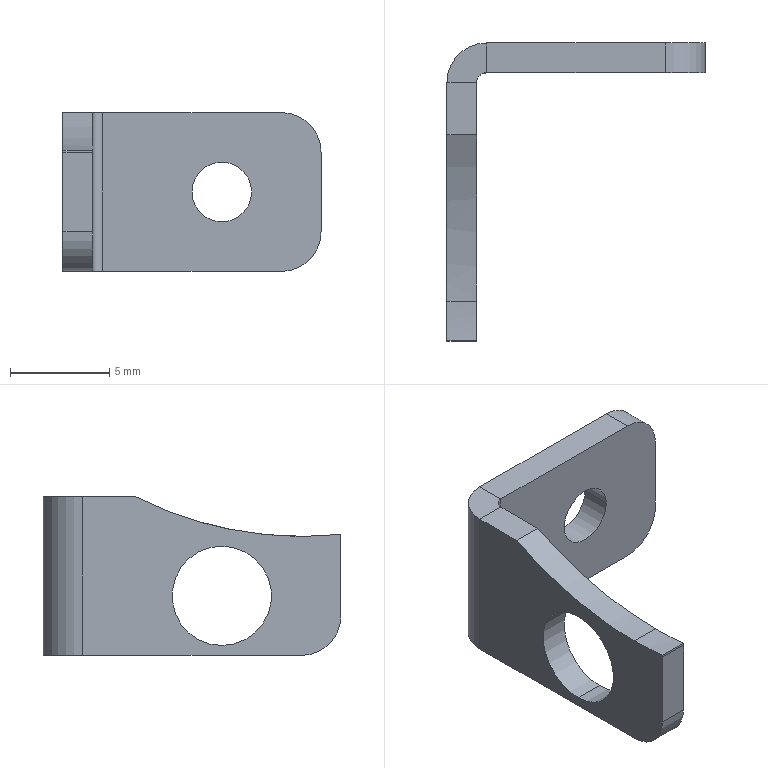Component | SolidWorks | ZHDJ-A0017-1 | 1 solid | 24 faces | box 13 x 15 x 8 mm | volume 245 mm3 | cylinder 12 | plane 12 | commonest cylinder face diameters 4 x5 37 x2 5 x2 3 x2 1 x1
STEP:
#1=COLOUR_RGB('',0.7922,0.8196,0.9333);
#2=FILL_AREA_STYLE_COLOUR('',#1);
#3=FILL_AREA_STYLE('',(#2));
#4=SURFACE_STYLE_FILL_AREA(#3);
#5=SURFACE_SIDE_STYLE('',(#4));
#6=SURFACE_STYLE_USAGE(.BOTH.,#5);
#7=PRESENTATION_STYLE_ASSIGNMENT((#6));
#8=CARTESIAN_POINT('',(0.2559,-0.07863,6.874));
#9=VERTEX_POINT('',#8);
#10=CARTESIAN_POINT('',(0.2559,0.,6.87));
#11=VERTEX_POINT('',#10);
#12=CARTESIAN_POINT('',(0.2559,0.,7.598));
#13=DIRECTION('',(1.,0.,-0.));
#14=DIRECTION('',(0.,-0.,1.));
#15=AXIS2_PLACEMENT_3D('',#12,#13,#14);
#16=CIRCLE('',#15,0.7283);
#17=EDGE_CURVE('',#9,#11,#16,.T.);
#18=ORIENTED_EDGE('',*,*,#17,.T.);
#19=CARTESIAN_POINT('',(0.1969,0.,6.87));
#20=VERTEX_POINT('',#19);
#21=CARTESIAN_POINT('',(0.7087,0.,6.87));
#22=DIRECTION('',(-1.,-0.,0.));
#23=VECTOR('',#22,39.37);
#24=LINE('',#21,#23);
#25=EDGE_CURVE('',#11,#20,#24,.T.);
#26=ORIENTED_EDGE('',*,*,#25,.T.);
#27=CARTESIAN_POINT('',(0.1969,-0.07862,6.874));
#28=VERTEX_POINT('',#27);
#29=CARTESIAN_POINT('',(0.1969,0.,6.87));
#30=CARTESIAN_POINT('',(0.1968,-0.02626,6.87));
#31=CARTESIAN_POINT('',(0.1968,-0.05252,6.872));
#32=CARTESIAN_POINT('',(0.1969,-0.07862,6.874));
#33=B_SPLINE_CURVE_WITH_KNOTS('',3,(#29,#30,#31,#32),.UNSPECIFIED.,.F.,.F.,(4,4),(0.8127,1.),.UNSPECIFIED.);
#34=EDGE_CURVE('',#20,#28,#33,.T.);
#35=ORIENTED_EDGE('',*,*,#34,.T.);
#36=CARTESIAN_POINT('',(0.4528,-0.07863,6.874));
#37=DIRECTION('',(1.,0.,-0.));
#38=VECTOR('',#37,39.37);
#39=LINE('',#36,#38);
#40=EDGE_CURVE('',#28,#9,#39,.T.);
#41=ORIENTED_EDGE('',*,*,#40,.T.);
#42=EDGE_LOOP('',(#18,#26,#35,#41));
#43=FACE_OUTER_BOUND('',#42,.T.);
#44=CARTESIAN_POINT('',(0.7087,0.,7.598));
#45=DIRECTION('',(-1.,-0.,0.));
#46=DIRECTION('',(0.,0.,-1.));
#47=AXIS2_PLACEMENT_3D('',#44,#45,#46);
#48=CYLINDRICAL_SURFACE('',#47,0.7283);
#49=ADVANCED_FACE('',(#43),#48,.F.);
#50=CARTESIAN_POINT('',(0.2559,0.1575,6.654));
#51=VERTEX_POINT('',#50);
#52=CARTESIAN_POINT('',(0.2559,0.1575,6.85));
#53=VERTEX_POINT('',#52);
#54=CARTESIAN_POINT('',(0.2559,0.1575,6.752));
#55=DIRECTION('',(1.,0.,-0.));
#56=DIRECTION('',(0.,0.,1.));
#57=AXIS2_PLACEMENT_3D('',#54,#55,#56);
#58=CIRCLE('',#57,0.09843);
#59=EDGE_CURVE('',#51,#53,#58,.T.);
#60=ORIENTED_EDGE('',*,*,#59,.T.);
#61=CARTESIAN_POINT('',(0.1969,0.1575,6.85));
#62=VERTEX_POINT('',#61);
#63=CARTESIAN_POINT('',(0.5906,0.1575,6.85));
#64=DIRECTION('',(-1.,-0.,0.));
#65=VECTOR('',#64,39.37);
#66=LINE('',#63,#65);
#67=EDGE_CURVE('',#53,#62,#66,.T.);
#68=ORIENTED_EDGE('',*,*,#67,.T.);
#69=CARTESIAN_POINT('',(0.1969,0.1575,6.654));
#70=VERTEX_POINT('',#69);
#71=CARTESIAN_POINT('',(0.1969,0.1575,6.752));
#72=DIRECTION('',(-1.,-0.,0.));
#73=DIRECTION('',(0.,0.,-1.));
#74=AXIS2_PLACEMENT_3D('',#71,#72,#73);
#75=CIRCLE('',#74,0.09843);
#76=EDGE_CURVE('',#62,#70,#75,.T.);
#77=ORIENTED_EDGE('',*,*,#76,.T.);
#78=CARTESIAN_POINT('',(0.5906,0.1575,6.654));
#79=DIRECTION('',(-1.,-0.,0.));
#80=VECTOR('',#79,39.37);
#81=LINE('',#78,#80);
#82=EDGE_CURVE('',#51,#70,#81,.T.);
#83=ORIENTED_EDGE('',*,*,#82,.F.);
#84=EDGE_LOOP('',(#60,#68,#77,#83));
#85=FACE_OUTER_BOUND('',#84,.T.);
#86=CARTESIAN_POINT('',(0.5906,0.1575,6.752));
#87=DIRECTION('',(-1.,-0.,0.));
#88=DIRECTION('',(0.,0.,-1.));
#89=AXIS2_PLACEMENT_3D('',#86,#87,#88);
#90=CYLINDRICAL_SURFACE('',#89,0.09843);
#91=ADVANCED_FACE('',(#85),#90,.F.);
#92=CARTESIAN_POINT('',(0.5709,0.5118,6.791));
#93=VERTEX_POINT('',#92);
#94=CARTESIAN_POINT('',(0.4528,0.5118,6.791));
#95=VERTEX_POINT('',#94);
#96=CARTESIAN_POINT('',(0.5118,0.5118,6.791));
#97=DIRECTION('',(0.,-1.,0.));
#98=DIRECTION('',(-1.,0.,0.));
#99=AXIS2_PLACEMENT_3D('',#96,#97,#98);
#100=CIRCLE('',#99,0.05906);
#101=EDGE_CURVE('',#93,#95,#100,.T.);
#102=ORIENTED_EDGE('',*,*,#101,.F.);
#103=CARTESIAN_POINT('',(0.5709,0.4528,6.791));
#104=VERTEX_POINT('',#103);
#105=CARTESIAN_POINT('',(0.5709,0.8465,6.791));
#106=DIRECTION('',(0.,-1.,0.));
#107=VECTOR('',#106,39.37);
#108=LINE('',#105,#107);
#109=EDGE_CURVE('',#93,#104,#108,.T.);
#110=ORIENTED_EDGE('',*,*,#109,.T.);
#111=CARTESIAN_POINT('',(0.4528,0.4528,6.791));
#112=VERTEX_POINT('',#111);
#113=CARTESIAN_POINT('',(0.5118,0.4528,6.791));
#114=DIRECTION('',(0.,-1.,0.));
#115=DIRECTION('',(-1.,0.,0.));
#116=AXIS2_PLACEMENT_3D('',#113,#114,#115);
#117=CIRCLE('',#116,0.05906);
#118=EDGE_CURVE('',#104,#112,#117,.T.);
#119=ORIENTED_EDGE('',*,*,#118,.T.);
#120=CARTESIAN_POINT('',(0.4528,0.8465,6.791));
#121=DIRECTION('',(0.,-1.,0.));
#122=VECTOR('',#121,39.37);
#123=LINE('',#120,#122);
#124=EDGE_CURVE('',#95,#112,#123,.T.);
#125=ORIENTED_EDGE('',*,*,#124,.F.);
#126=EDGE_LOOP('',(#102,#110,#119,#125));
#127=FACE_OUTER_BOUND('',#126,.T.);
#128=CARTESIAN_POINT('',(0.5118,0.8465,6.791));
#129=DIRECTION('',(0.,-1.,0.));
#130=DIRECTION('',(-1.,0.,0.));
#131=AXIS2_PLACEMENT_3D('',#128,#129,#130);
#132=CYLINDRICAL_SURFACE('',#131,0.05906);
#133=ADVANCED_FACE('',(#127),#132,.F.);
#134=CARTESIAN_POINT('',(0.1969,0.1575,6.752));
#135=DIRECTION('',(-1.,-0.,0.));
#136=DIRECTION('',(0.,0.,-1.));
#137=AXIS2_PLACEMENT_3D('',#134,#135,#136);
#138=CIRCLE('',#137,0.09843);
#139=EDGE_CURVE('',#70,#62,#138,.T.);
#140=ORIENTED_EDGE('',*,*,#139,.F.);
#141=ORIENTED_EDGE('',*,*,#76,.F.);
#142=EDGE_LOOP('',(#140,#141));
#143=FACE_BOUND('',#142,.T.);
#144=CARTESIAN_POINT('',(0.1969,0.3295,6.949));
#145=VERTEX_POINT('',#144);
#146=CARTESIAN_POINT('',(0.1969,0.3295,6.949));
#147=CARTESIAN_POINT('',(0.1968,0.2786,6.923));
#148=CARTESIAN_POINT('',(0.1968,0.2248,6.903));
#149=CARTESIAN_POINT('',(0.1968,0.1139,6.877));
#150=CARTESIAN_POINT('',(0.1968,0.05698,6.87));
#151=CARTESIAN_POINT('',(0.1969,0.,6.87));
#152=B_SPLINE_CURVE_WITH_KNOTS('',3,(#146,#147,#148,#149,#150,#151),.UNSPECIFIED.,.F.,.F.,(4,2,4),(0.,0.4064,0.8127),.UNSPECIFIED.);
#153=EDGE_CURVE('',#145,#20,#152,.T.);
#154=ORIENTED_EDGE('',*,*,#153,.F.);
#155=CARTESIAN_POINT('',(0.1969,0.4331,6.949));
#156=VERTEX_POINT('',#155);
#157=CARTESIAN_POINT('',(0.1969,0.4528,6.949));
#158=DIRECTION('',(-0.,1.,0.));
#159=VECTOR('',#158,39.37);
#160=LINE('',#157,#159);
#161=EDGE_CURVE('',#145,#156,#160,.T.);
#162=ORIENTED_EDGE('',*,*,#161,.T.);
#163=CARTESIAN_POINT('',(0.1969,0.4331,6.634));
#164=VERTEX_POINT('',#163);
#165=CARTESIAN_POINT('',(0.1969,0.4331,6.949));
#166=DIRECTION('',(0.,-0.,1.));
#167=VECTOR('',#166,39.37);
#168=LINE('',#165,#167);
#169=EDGE_CURVE('',#164,#156,#168,.T.);
#170=ORIENTED_EDGE('',*,*,#169,.F.);
#171=CARTESIAN_POINT('',(0.1969,0.,6.634));
#172=VERTEX_POINT('',#171);
#173=CARTESIAN_POINT('',(0.1969,0.4528,6.634));
#174=DIRECTION('',(0.,-1.,0.));
#175=VECTOR('',#174,39.37);
#176=LINE('',#173,#175);
#177=EDGE_CURVE('',#164,#172,#176,.T.);
#178=ORIENTED_EDGE('',*,*,#177,.T.);
#179=CARTESIAN_POINT('',(0.1969,-0.07874,6.713));
#180=VERTEX_POINT('',#179);
#181=CARTESIAN_POINT('',(0.1969,0.,6.713));
#182=DIRECTION('',(-1.,-0.,0.));
#183=DIRECTION('',(0.,-0.,1.));
#184=AXIS2_PLACEMENT_3D('',#181,#182,#183);
#185=CIRCLE('',#184,0.07874);
#186=EDGE_CURVE('',#172,#180,#185,.T.);
#187=ORIENTED_EDGE('',*,*,#186,.T.);
#188=CARTESIAN_POINT('',(0.1969,-0.07874,6.87));
#189=VERTEX_POINT('',#188);
#190=CARTESIAN_POINT('',(0.1969,-0.07874,6.791));
#191=DIRECTION('',(0.,-0.,1.));
#192=VECTOR('',#191,39.37);
#193=LINE('',#190,#192);
#194=EDGE_CURVE('',#180,#189,#193,.T.);
#195=ORIENTED_EDGE('',*,*,#194,.T.);
#196=CARTESIAN_POINT('',(0.1969,0.,6.87));
#197=DIRECTION('',(-1.,-0.,0.));
#198=DIRECTION('',(0.,0.,1.));
#199=AXIS2_PLACEMENT_3D('',#196,#197,#198);
#200=CIRCLE('',#199,0.07874);
#201=EDGE_CURVE('',#189,#28,#200,.T.);
#202=ORIENTED_EDGE('',*,*,#201,.T.);
#203=ORIENTED_EDGE('',*,*,#34,.F.);
#204=EDGE_LOOP('',(#154,#162,#170,#178,#187,#195,#202,#203));
#205=FACE_OUTER_BOUND('',#204,.T.);
#206=CARTESIAN_POINT('',(0.1969,0.4528,6.791));
#207=DIRECTION('',(1.,0.,-0.));
#208=DIRECTION('',(0.,-0.,1.));
#209=AXIS2_PLACEMENT_3D('',#206,#207,#208);
#210=PLANE('',#209);
#211=ADVANCED_FACE('',(#143,#205),#210,.F.);
#212=CARTESIAN_POINT('',(0.5118,0.5118,6.791));
#213=DIRECTION('',(0.,-1.,0.));
#214=DIRECTION('',(-1.,0.,0.));
#215=AXIS2_PLACEMENT_3D('',#212,#213,#214);
#216=CIRCLE('',#215,0.05906);
#217=EDGE_CURVE('',#95,#93,#216,.T.);
#218=ORIENTED_EDGE('',*,*,#217,.T.);
#219=ORIENTED_EDGE('',*,*,#101,.T.);
#220=EDGE_LOOP('',(#218,#219));
#221=FACE_BOUND('',#220,.T.);
#222=CARTESIAN_POINT('',(0.7087,0.5118,6.713));
#223=VERTEX_POINT('',#222);
#224=CARTESIAN_POINT('',(0.7087,0.5118,6.87));
#225=VERTEX_POINT('',#224);
#226=CARTESIAN_POINT('',(0.7087,0.5118,6.634));
#227=DIRECTION('',(0.,-0.,1.));
#228=VECTOR('',#227,39.37);
#229=LINE('',#226,#228);
#230=EDGE_CURVE('',#223,#225,#229,.T.);
#231=ORIENTED_EDGE('',*,*,#230,.F.);
#232=CARTESIAN_POINT('',(0.6299,0.5118,6.634));
#233=VERTEX_POINT('',#232);
#234=CARTESIAN_POINT('',(0.6299,0.5118,6.713));
#235=DIRECTION('',(-0.,1.,0.));
#236=DIRECTION('',(-1.,0.,0.));
#237=AXIS2_PLACEMENT_3D('',#234,#235,#236);
#238=CIRCLE('',#237,0.07874);
#239=EDGE_CURVE('',#223,#233,#238,.T.);
#240=ORIENTED_EDGE('',*,*,#239,.T.);
#241=CARTESIAN_POINT('',(0.2756,0.5118,6.634));
#242=VERTEX_POINT('',#241);
#243=CARTESIAN_POINT('',(0.1969,0.5118,6.634));
#244=DIRECTION('',(1.,0.,-0.));
#245=VECTOR('',#244,39.37);
#246=LINE('',#243,#245);
#247=EDGE_CURVE('',#242,#233,#246,.T.);
#248=ORIENTED_EDGE('',*,*,#247,.F.);
#249=CARTESIAN_POINT('',(0.2756,0.5118,6.949));
#250=VERTEX_POINT('',#249);
#251=CARTESIAN_POINT('',(0.2756,0.5118,6.634));
#252=DIRECTION('',(0.,-0.,1.));
#253=VECTOR('',#252,39.37);
#254=LINE('',#251,#253);
#255=EDGE_CURVE('',#242,#250,#254,.T.);
#256=ORIENTED_EDGE('',*,*,#255,.T.);
#257=CARTESIAN_POINT('',(0.6299,0.5118,6.949));
#258=VERTEX_POINT('',#257);
#259=CARTESIAN_POINT('',(0.1969,0.5118,6.949));
#260=DIRECTION('',(1.,0.,-0.));
#261=VECTOR('',#260,39.37);
#262=LINE('',#259,#261);
#263=EDGE_CURVE('',#250,#258,#262,.T.);
#264=ORIENTED_EDGE('',*,*,#263,.T.);
#265=CARTESIAN_POINT('',(0.6299,0.5118,6.87));
#266=DIRECTION('',(-0.,1.,0.));
#267=DIRECTION('',(-1.,0.,0.));
#268=AXIS2_PLACEMENT_3D('',#265,#266,#267);
#269=CIRCLE('',#268,0.07874);
#270=EDGE_CURVE('',#258,#225,#269,.T.);
#271=ORIENTED_EDGE('',*,*,#270,.T.);
#272=EDGE_LOOP('',(#231,#240,#248,#256,#264,#271));
#273=FACE_OUTER_BOUND('',#272,.T.);
#274=CARTESIAN_POINT('',(0.1969,0.5118,6.634));
#275=DIRECTION('',(0.,-1.,-0.));
#276=DIRECTION('',(-1.,-0.,0.));
#277=AXIS2_PLACEMENT_3D('',#274,#275,#276);
#278=PLANE('',#277);
#279=ADVANCED_FACE('',(#221,#273),#278,.F.);
#280=CARTESIAN_POINT('',(0.5118,0.4528,6.791));
#281=DIRECTION('',(0.,-1.,0.));
#282=DIRECTION('',(-1.,0.,0.));
#283=AXIS2_PLACEMENT_3D('',#280,#281,#282);
#284=CIRCLE('',#283,0.05906);
#285=EDGE_CURVE('',#112,#104,#284,.T.);
#286=ORIENTED_EDGE('',*,*,#285,.F.);
#287=ORIENTED_EDGE('',*,*,#118,.F.);
#288=EDGE_LOOP('',(#286,#287));
#289=FACE_BOUND('',#288,.T.);
#290=CARTESIAN_POINT('',(0.2756,0.4528,6.634));
#291=VERTEX_POINT('',#290);
#292=CARTESIAN_POINT('',(0.6299,0.4528,6.634));
#293=VERTEX_POINT('',#292);
#294=CARTESIAN_POINT('',(0.1969,0.4528,6.634));
#295=DIRECTION('',(1.,0.,-0.));
#296=VECTOR('',#295,39.37);
#297=LINE('',#294,#296);
#298=EDGE_CURVE('',#291,#293,#297,.T.);
#299=ORIENTED_EDGE('',*,*,#298,.T.);
#300=CARTESIAN_POINT('',(0.7087,0.4528,6.713));
#301=VERTEX_POINT('',#300);
#302=CARTESIAN_POINT('',(0.6299,0.4528,6.713));
#303=DIRECTION('',(0.,-1.,0.));
#304=DIRECTION('',(-1.,0.,0.));
#305=AXIS2_PLACEMENT_3D('',#302,#303,#304);
#306=CIRCLE('',#305,0.07874);
#307=EDGE_CURVE('',#293,#301,#306,.T.);
#308=ORIENTED_EDGE('',*,*,#307,.T.);
#309=CARTESIAN_POINT('',(0.7087,0.4528,6.87));
#310=VERTEX_POINT('',#309);
#311=CARTESIAN_POINT('',(0.7087,0.4528,6.634));
#312=DIRECTION('',(0.,-0.,1.));
#313=VECTOR('',#312,39.37);
#314=LINE('',#311,#313);
#315=EDGE_CURVE('',#301,#310,#314,.T.);
#316=ORIENTED_EDGE('',*,*,#315,.T.);
#317=CARTESIAN_POINT('',(0.6299,0.4528,6.949));
#318=VERTEX_POINT('',#317);
#319=CARTESIAN_POINT('',(0.6299,0.4528,6.87));
#320=DIRECTION('',(0.,-1.,0.));
#321=DIRECTION('',(-1.,0.,0.));
#322=AXIS2_PLACEMENT_3D('',#319,#320,#321);
#323=CIRCLE('',#322,0.07874);
#324=EDGE_CURVE('',#310,#318,#323,.T.);
#325=ORIENTED_EDGE('',*,*,#324,.T.);
#326=CARTESIAN_POINT('',(0.2756,0.4528,6.949));
#327=VERTEX_POINT('',#326);
#328=CARTESIAN_POINT('',(0.1969,0.4528,6.949));
#329=DIRECTION('',(1.,0.,-0.));
#330=VECTOR('',#329,39.37);
#331=LINE('',#328,#330);
#332=EDGE_CURVE('',#327,#318,#331,.T.);
#333=ORIENTED_EDGE('',*,*,#332,.F.);
#334=CARTESIAN_POINT('',(0.2756,0.4528,6.634));
#335=DIRECTION('',(0.,-0.,1.));
#336=VECTOR('',#335,39.37);
#337=LINE('',#334,#336);
#338=EDGE_CURVE('',#291,#327,#337,.T.);
#339=ORIENTED_EDGE('',*,*,#338,.F.);
#340=EDGE_LOOP('',(#299,#308,#316,#325,#333,#339));
#341=FACE_OUTER_BOUND('',#340,.T.);
#342=CARTESIAN_POINT('',(0.1969,0.4528,6.634));
#343=DIRECTION('',(0.,-1.,-0.));
#344=DIRECTION('',(-1.,-0.,0.));
#345=AXIS2_PLACEMENT_3D('',#342,#343,#344);
#346=PLANE('',#345);
#347=ADVANCED_FACE('',(#289,#341),#346,.T.);
#348=ORIENTED_EDGE('',*,*,#247,.T.);
#349=CARTESIAN_POINT('',(0.6299,0.4528,6.634));
#350=DIRECTION('',(0.,-1.,0.));
#351=VECTOR('',#350,39.37);
#352=LINE('',#349,#351);
#353=EDGE_CURVE('',#233,#293,#352,.T.);
#354=ORIENTED_EDGE('',*,*,#353,.T.);
#355=ORIENTED_EDGE('',*,*,#298,.F.);
#356=CARTESIAN_POINT('',(0.2756,0.4528,6.634));
#357=DIRECTION('',(-0.,1.,0.));
#358=VECTOR('',#357,39.37);
#359=LINE('',#356,#358);
#360=EDGE_CURVE('',#291,#242,#359,.T.);
#361=ORIENTED_EDGE('',*,*,#360,.T.);
#362=EDGE_LOOP('',(#348,#354,#355,#361));
#363=FACE_OUTER_BOUND('',#362,.T.);
#364=CARTESIAN_POINT('',(0.1969,0.4528,6.634));
#365=DIRECTION('',(0.,-0.,1.));
#366=DIRECTION('',(-1.,-0.,0.));
#367=AXIS2_PLACEMENT_3D('',#364,#365,#366);
#368=PLANE('',#367);
#369=ADVANCED_FACE('',(#363),#368,.F.);
#370=ORIENTED_EDGE('',*,*,#315,.F.);
#371=CARTESIAN_POINT('',(0.7087,0.5118,6.713));
#372=DIRECTION('',(-0.,1.,0.));
#373=VECTOR('',#372,39.37);
#374=LINE('',#371,#373);
#375=EDGE_CURVE('',#301,#223,#374,.T.);
#376=ORIENTED_EDGE('',*,*,#375,.T.);
#377=ORIENTED_EDGE('',*,*,#230,.T.);
#378=CARTESIAN_POINT('',(0.7087,0.4528,6.87));
#379=DIRECTION('',(0.,-1.,0.));
#380=VECTOR('',#379,39.37);
#381=LINE('',#378,#380);
#382=EDGE_CURVE('',#225,#310,#381,.T.);
#383=ORIENTED_EDGE('',*,*,#382,.T.);
#384=EDGE_LOOP('',(#370,#376,#377,#383));
#385=FACE_OUTER_BOUND('',#384,.T.);
#386=CARTESIAN_POINT('',(0.7087,0.4528,6.634));
#387=DIRECTION('',(1.,0.,-0.));
#388=DIRECTION('',(0.,-0.,1.));
#389=AXIS2_PLACEMENT_3D('',#386,#387,#388);
#390=PLANE('',#389);
#391=ADVANCED_FACE('',(#385),#390,.T.);
#392=ORIENTED_EDGE('',*,*,#332,.T.);
#393=CARTESIAN_POINT('',(0.6299,0.4528,6.949));
#394=DIRECTION('',(-0.,1.,0.));
#395=VECTOR('',#394,39.37);
#396=LINE('',#393,#395);
#397=EDGE_CURVE('',#318,#258,#396,.T.);
#398=ORIENTED_EDGE('',*,*,#397,.T.);
#399=ORIENTED_EDGE('',*,*,#263,.F.);
#400=CARTESIAN_POINT('',(0.2756,0.4528,6.949));
#401=DIRECTION('',(-0.,1.,0.));
#402=VECTOR('',#401,39.37);
#403=LINE('',#400,#402);
#404=EDGE_CURVE('',#327,#250,#403,.T.);
#405=ORIENTED_EDGE('',*,*,#404,.F.);
#406=EDGE_LOOP('',(#392,#398,#399,#405));
#407=FACE_OUTER_BOUND('',#406,.T.);
#408=CARTESIAN_POINT('',(0.1969,0.4528,6.949));
#409=DIRECTION('',(0.,-0.,1.));
#410=DIRECTION('',(-1.,-0.,0.));
#411=AXIS2_PLACEMENT_3D('',#408,#409,#410);
#412=PLANE('',#411);
#413=ADVANCED_FACE('',(#407),#412,.T.);
#414=CARTESIAN_POINT('',(0.2559,0.4331,6.949));
#415=VERTEX_POINT('',#414);
#416=CARTESIAN_POINT('',(0.1969,0.4331,6.949));
#417=DIRECTION('',(-1.,-0.,0.));
#418=VECTOR('',#417,39.37);
#419=LINE('',#416,#418);
#420=EDGE_CURVE('',#415,#156,#419,.T.);
#421=ORIENTED_EDGE('',*,*,#420,.F.);
#422=CARTESIAN_POINT('',(0.2756,0.4331,6.949));
#423=DIRECTION('',(0.,-0.,1.));
#424=DIRECTION('',(1.,0.,0.));
#425=AXIS2_PLACEMENT_3D('',#422,#423,#424);
#426=CIRCLE('',#425,0.01969);
#427=EDGE_CURVE('',#327,#415,#426,.T.);
#428=ORIENTED_EDGE('',*,*,#427,.F.);
#429=ORIENTED_EDGE('',*,*,#404,.T.);
#430=CARTESIAN_POINT('',(0.2756,0.4331,6.949));
#431=DIRECTION('',(0.,-0.,1.));
#432=DIRECTION('',(1.,-0.,0.));
#433=AXIS2_PLACEMENT_3D('',#430,#431,#432);
#434=CIRCLE('',#433,0.07874);
#435=EDGE_CURVE('',#250,#156,#434,.T.);
#436=ORIENTED_EDGE('',*,*,#435,.T.);
#437=EDGE_LOOP('',(#421,#428,#429,#436));
#438=FACE_OUTER_BOUND('',#437,.T.);
#439=CARTESIAN_POINT('',(0.2756,0.4331,6.949));
#440=DIRECTION('',(0.,-0.,1.));
#441=DIRECTION('',(-1.,-0.,0.));
#442=AXIS2_PLACEMENT_3D('',#439,#440,#441);
#443=PLANE('',#442);
#444=ADVANCED_FACE('',(#438),#443,.T.);
#445=CARTESIAN_POINT('',(0.2559,0.4331,6.634));
#446=VERTEX_POINT('',#445);
#447=CARTESIAN_POINT('',(0.2756,0.4331,6.634));
#448=DIRECTION('',(-0.,0.,-1.));
#449=DIRECTION('',(1.,0.,0.));
#450=AXIS2_PLACEMENT_3D('',#447,#448,#449);
#451=CIRCLE('',#450,0.01969);
#452=EDGE_CURVE('',#446,#291,#451,.T.);
#453=ORIENTED_EDGE('',*,*,#452,.F.);
#454=CARTESIAN_POINT('',(0.2559,0.4331,6.634));
#455=DIRECTION('',(-1.,-0.,0.));
#456=VECTOR('',#455,39.37);
#457=LINE('',#454,#456);
#458=EDGE_CURVE('',#446,#164,#457,.T.);
#459=ORIENTED_EDGE('',*,*,#458,.T.);
#460=CARTESIAN_POINT('',(0.2756,0.4331,6.634));
#461=DIRECTION('',(-0.,0.,-1.));
#462=DIRECTION('',(1.,0.,0.));
#463=AXIS2_PLACEMENT_3D('',#460,#461,#462);
#464=CIRCLE('',#463,0.07874);
#465=EDGE_CURVE('',#164,#242,#464,.T.);
#466=ORIENTED_EDGE('',*,*,#465,.T.);
#467=ORIENTED_EDGE('',*,*,#360,.F.);
#468=EDGE_LOOP('',(#453,#459,#466,#467));
#469=FACE_OUTER_BOUND('',#468,.T.);
#470=CARTESIAN_POINT('',(0.2756,0.4331,6.634));
#471=DIRECTION('',(0.,-0.,1.));
#472=DIRECTION('',(-1.,-0.,0.));
#473=AXIS2_PLACEMENT_3D('',#470,#471,#472);
#474=PLANE('',#473);
#475=ADVANCED_FACE('',(#469),#474,.F.);
#476=ORIENTED_EDGE('',*,*,#255,.F.);
#477=ORIENTED_EDGE('',*,*,#465,.F.);
#478=ORIENTED_EDGE('',*,*,#169,.T.);
#479=ORIENTED_EDGE('',*,*,#435,.F.);
#480=EDGE_LOOP('',(#476,#477,#478,#479));
#481=FACE_OUTER_BOUND('',#480,.T.);
#482=CARTESIAN_POINT('',(0.2756,0.4331,6.634));
#483=DIRECTION('',(-0.,0.,-1.));
#484=DIRECTION('',(-1.,0.,0.));
#485=AXIS2_PLACEMENT_3D('',#482,#483,#484);
#486=CYLINDRICAL_SURFACE('',#485,0.07874);
#487=ADVANCED_FACE('',(#481),#486,.T.);
#488=ORIENTED_EDGE('',*,*,#338,.T.);
#489=ORIENTED_EDGE('',*,*,#427,.T.);
#490=CARTESIAN_POINT('',(0.2559,0.4331,6.949));
#491=DIRECTION('',(-0.,0.,-1.));
#492=VECTOR('',#491,39.37);
#493=LINE('',#490,#492);
#494=EDGE_CURVE('',#415,#446,#493,.T.);
#495=ORIENTED_EDGE('',*,*,#494,.T.);
#496=ORIENTED_EDGE('',*,*,#452,.T.);
#497=EDGE_LOOP('',(#488,#489,#495,#496));
#498=FACE_OUTER_BOUND('',#497,.T.);
#499=CARTESIAN_POINT('',(0.2756,0.4331,6.634));
#500=DIRECTION('',(-0.,0.,-1.));
#501=DIRECTION('',(-1.,0.,0.));
#502=AXIS2_PLACEMENT_3D('',#499,#500,#501);
#503=CYLINDRICAL_SURFACE('',#502,0.01969);
#504=ADVANCED_FACE('',(#498),#503,.F.);
#505=CARTESIAN_POINT('',(0.2559,0.,6.634));
#506=VERTEX_POINT('',#505);
#507=CARTESIAN_POINT('',(0.2559,-0.07874,6.634));
#508=DIRECTION('',(0.,-1.,0.));
#509=VECTOR('',#508,39.37);
#510=LINE('',#507,#509);
#511=EDGE_CURVE('',#446,#506,#510,.T.);
#512=ORIENTED_EDGE('',*,*,#511,.T.);
#513=CARTESIAN_POINT('',(0.1969,0.,6.634));
#514=DIRECTION('',(-1.,-0.,0.));
#515=VECTOR('',#514,39.37);
#516=LINE('',#513,#515);
#517=EDGE_CURVE('',#506,#172,#516,.T.);
#518=ORIENTED_EDGE('',*,*,#517,.T.);
#519=ORIENTED_EDGE('',*,*,#177,.F.);
#520=ORIENTED_EDGE('',*,*,#458,.F.);
#521=EDGE_LOOP('',(#512,#518,#519,#520));
#522=FACE_OUTER_BOUND('',#521,.T.);
#523=CARTESIAN_POINT('',(0.1969,-0.07874,6.634));
#524=DIRECTION('',(0.,0.,1.));
#525=DIRECTION('',(-0.,1.,-0.));
#526=AXIS2_PLACEMENT_3D('',#523,#524,#525);
#527=PLANE('',#526);
#528=ADVANCED_FACE('',(#522),#527,.F.);
#529=ORIENTED_EDGE('',*,*,#161,.F.);
#530=CARTESIAN_POINT('',(0.2559,0.3294,6.949));
#531=VERTEX_POINT('',#530);
#532=CARTESIAN_POINT('',(0.7087,0.3294,6.949));
#533=DIRECTION('',(1.,0.,-0.));
#534=VECTOR('',#533,39.37);
#535=LINE('',#532,#534);
#536=EDGE_CURVE('',#145,#531,#535,.T.);
#537=ORIENTED_EDGE('',*,*,#536,.T.);
#538=CARTESIAN_POINT('',(0.2559,0.4528,6.949));
#539=DIRECTION('',(-0.,1.,0.));
#540=VECTOR('',#539,39.37);
#541=LINE('',#538,#540);
#542=EDGE_CURVE('',#531,#415,#541,.T.);
#543=ORIENTED_EDGE('',*,*,#542,.T.);
#544=ORIENTED_EDGE('',*,*,#420,.T.);
#545=EDGE_LOOP('',(#529,#537,#543,#544));
#546=FACE_OUTER_BOUND('',#545,.T.);
#547=CARTESIAN_POINT('',(0.1969,0.4528,6.949));
#548=DIRECTION('',(-0.,0.,-1.));
#549=DIRECTION('',(1.,0.,-0.));
#550=AXIS2_PLACEMENT_3D('',#547,#548,#549);
#551=PLANE('',#550);
#552=ADVANCED_FACE('',(#546),#551,.F.);
#553=ORIENTED_EDGE('',*,*,#17,.F.);
#554=CARTESIAN_POINT('',(0.2559,-0.07874,6.87));
#555=VERTEX_POINT('',#554);
#556=CARTESIAN_POINT('',(0.2559,0.,6.87));
#557=DIRECTION('',(1.,0.,-0.));
#558=DIRECTION('',(0.,-0.,1.));
#559=AXIS2_PLACEMENT_3D('',#556,#557,#558);
#560=CIRCLE('',#559,0.07874);
#561=EDGE_CURVE('',#9,#555,#560,.T.);
#562=ORIENTED_EDGE('',*,*,#561,.T.);
#563=CARTESIAN_POINT('',(0.2559,-0.07874,6.713));
#564=VERTEX_POINT('',#563);
#565=CARTESIAN_POINT('',(0.2559,-0.07874,6.949));
#566=DIRECTION('',(0.,-0.,1.));
#567=VECTOR('',#566,39.37);
#568=LINE('',#565,#567);
#569=EDGE_CURVE('',#564,#555,#568,.T.);
#570=ORIENTED_EDGE('',*,*,#569,.F.);
#571=CARTESIAN_POINT('',(0.2559,0.,6.713));
#572=DIRECTION('',(1.,0.,-0.));
#573=DIRECTION('',(0.,-0.,1.));
#574=AXIS2_PLACEMENT_3D('',#571,#572,#573);
#575=CIRCLE('',#574,0.07874);
#576=EDGE_CURVE('',#564,#506,#575,.T.);
#577=ORIENTED_EDGE('',*,*,#576,.T.);
#578=ORIENTED_EDGE('',*,*,#511,.F.);
#579=ORIENTED_EDGE('',*,*,#494,.F.);
#580=ORIENTED_EDGE('',*,*,#542,.F.);
#581=CARTESIAN_POINT('',(0.2559,0.,7.598));
#582=DIRECTION('',(1.,0.,-0.));
#583=DIRECTION('',(0.,-0.,1.));
#584=AXIS2_PLACEMENT_3D('',#581,#582,#583);
#585=CIRCLE('',#584,0.7283);
#586=EDGE_CURVE('',#11,#531,#585,.T.);
#587=ORIENTED_EDGE('',*,*,#586,.F.);
#588=EDGE_LOOP('',(#553,#562,#570,#577,#578,#579,#580,#587));
#589=FACE_OUTER_BOUND('',#588,.T.);
#590=ORIENTED_EDGE('',*,*,#59,.F.);
#591=CARTESIAN_POINT('',(0.2559,0.1575,6.752));
#592=DIRECTION('',(1.,0.,-0.));
#593=DIRECTION('',(0.,0.,1.));
#594=AXIS2_PLACEMENT_3D('',#591,#592,#593);
#595=CIRCLE('',#594,0.09843);
#596=EDGE_CURVE('',#53,#51,#595,.T.);
#597=ORIENTED_EDGE('',*,*,#596,.F.);
#598=EDGE_LOOP('',(#590,#597));
#599=FACE_BOUND('',#598,.T.);
#600=CARTESIAN_POINT('',(0.2559,0.4528,6.791));
#601=DIRECTION('',(1.,0.,-0.));
#602=DIRECTION('',(0.,-0.,1.));
#603=AXIS2_PLACEMENT_3D('',#600,#601,#602);
#604=PLANE('',#603);
#605=ADVANCED_FACE('',(#589,#599),#604,.T.);
#606=ORIENTED_EDGE('',*,*,#194,.F.);
#607=CARTESIAN_POINT('',(0.1969,-0.07874,6.713));
#608=DIRECTION('',(1.,0.,-0.));
#609=VECTOR('',#608,39.37);
#610=LINE('',#607,#609);
#611=EDGE_CURVE('',#180,#564,#610,.T.);
#612=ORIENTED_EDGE('',*,*,#611,.T.);
#613=ORIENTED_EDGE('',*,*,#569,.T.);
#614=CARTESIAN_POINT('',(0.1969,-0.07874,6.87));
#615=DIRECTION('',(-1.,-0.,0.));
#616=VECTOR('',#615,39.37);
#617=LINE('',#614,#616);
#618=EDGE_CURVE('',#555,#189,#617,.T.);
#619=ORIENTED_EDGE('',*,*,#618,.T.);
#620=EDGE_LOOP('',(#606,#612,#613,#619));
#621=FACE_OUTER_BOUND('',#620,.T.);
#622=CARTESIAN_POINT('',(0.1969,-0.07874,6.949));
#623=DIRECTION('',(-0.,1.,0.));
#624=DIRECTION('',(1.,0.,-0.));
#625=AXIS2_PLACEMENT_3D('',#622,#623,#624);
#626=PLANE('',#625);
#627=ADVANCED_FACE('',(#621),#626,.F.);
#628=ORIENTED_EDGE('',*,*,#307,.F.);
#629=ORIENTED_EDGE('',*,*,#353,.F.);
#630=ORIENTED_EDGE('',*,*,#239,.F.);
#631=ORIENTED_EDGE('',*,*,#375,.F.);
#632=EDGE_LOOP('',(#628,#629,#630,#631));
#633=FACE_OUTER_BOUND('',#632,.T.);
#634=CARTESIAN_POINT('',(0.6299,0.4528,6.713));
#635=DIRECTION('',(0.,-1.,0.));
#636=DIRECTION('',(-1.,0.,0.));
#637=AXIS2_PLACEMENT_3D('',#634,#635,#636);
#638=CYLINDRICAL_SURFACE('',#637,0.07874);
#639=ADVANCED_FACE('',(#633),#638,.T.);
#640=ORIENTED_EDGE('',*,*,#324,.F.);
#641=ORIENTED_EDGE('',*,*,#382,.F.);
#642=ORIENTED_EDGE('',*,*,#270,.F.);
#643=ORIENTED_EDGE('',*,*,#397,.F.);
#644=EDGE_LOOP('',(#640,#641,#642,#643));
#645=FACE_OUTER_BOUND('',#644,.T.);
#646=CARTESIAN_POINT('',(0.6299,0.4528,6.87));
#647=DIRECTION('',(-0.,1.,0.));
#648=DIRECTION('',(1.,0.,0.));
#649=AXIS2_PLACEMENT_3D('',#646,#647,#648);
#650=CYLINDRICAL_SURFACE('',#649,0.07874);
#651=ADVANCED_FACE('',(#645),#650,.T.);
#652=ORIENTED_EDGE('',*,*,#109,.F.);
#653=ORIENTED_EDGE('',*,*,#217,.F.);
#654=ORIENTED_EDGE('',*,*,#124,.T.);
#655=ORIENTED_EDGE('',*,*,#285,.T.);
#656=EDGE_LOOP('',(#652,#653,#654,#655));
#657=FACE_OUTER_BOUND('',#656,.T.);
#658=CARTESIAN_POINT('',(0.5118,0.8465,6.791));
#659=DIRECTION('',(0.,-1.,0.));
#660=DIRECTION('',(-1.,0.,0.));
#661=AXIS2_PLACEMENT_3D('',#658,#659,#660);
#662=CYLINDRICAL_SURFACE('',#661,0.05906);
#663=ADVANCED_FACE('',(#657),#662,.F.);
#664=ORIENTED_EDGE('',*,*,#67,.F.);
#665=ORIENTED_EDGE('',*,*,#596,.T.);
#666=ORIENTED_EDGE('',*,*,#82,.T.);
#667=ORIENTED_EDGE('',*,*,#139,.T.);
#668=EDGE_LOOP('',(#664,#665,#666,#667));
#669=FACE_OUTER_BOUND('',#668,.T.);
#670=CARTESIAN_POINT('',(0.5906,0.1575,6.752));
#671=DIRECTION('',(-1.,-0.,0.));
#672=DIRECTION('',(0.,0.,-1.));
#673=AXIS2_PLACEMENT_3D('',#670,#671,#672);
#674=CYLINDRICAL_SURFACE('',#673,0.09843);
#675=ADVANCED_FACE('',(#669),#674,.F.);
#676=ORIENTED_EDGE('',*,*,#186,.F.);
#677=ORIENTED_EDGE('',*,*,#517,.F.);
#678=ORIENTED_EDGE('',*,*,#576,.F.);
#679=ORIENTED_EDGE('',*,*,#611,.F.);
#680=EDGE_LOOP('',(#676,#677,#678,#679));
#681=FACE_OUTER_BOUND('',#680,.T.);
#682=CARTESIAN_POINT('',(0.1969,0.,6.713));
#683=DIRECTION('',(1.,0.,-0.));
#684=DIRECTION('',(0.,-0.,1.));
#685=AXIS2_PLACEMENT_3D('',#682,#683,#684);
#686=CYLINDRICAL_SURFACE('',#685,0.07874);
#687=ADVANCED_FACE('',(#681),#686,.T.);
#688=ORIENTED_EDGE('',*,*,#40,.F.);
#689=ORIENTED_EDGE('',*,*,#201,.F.);
#690=ORIENTED_EDGE('',*,*,#618,.F.);
#691=ORIENTED_EDGE('',*,*,#561,.F.);
#692=EDGE_LOOP('',(#688,#689,#690,#691));
#693=FACE_OUTER_BOUND('',#692,.T.);
#694=CARTESIAN_POINT('',(0.1969,0.,6.87));
#695=DIRECTION('',(1.,0.,-0.));
#696=DIRECTION('',(0.,-0.,1.));
#697=AXIS2_PLACEMENT_3D('',#694,#695,#696);
#698=CYLINDRICAL_SURFACE('',#697,0.07874);
#699=ADVANCED_FACE('',(#693),#698,.T.);
#700=ORIENTED_EDGE('',*,*,#25,.F.);
#701=ORIENTED_EDGE('',*,*,#586,.T.);
#702=ORIENTED_EDGE('',*,*,#536,.F.);
#703=ORIENTED_EDGE('',*,*,#153,.T.);
#704=EDGE_LOOP('',(#700,#701,#702,#703));
#705=FACE_OUTER_BOUND('',#704,.T.);
#706=CARTESIAN_POINT('',(0.7087,0.,7.598));
#707=DIRECTION('',(-1.,-0.,0.));
#708=DIRECTION('',(0.,0.,-1.));
#709=AXIS2_PLACEMENT_3D('',#706,#707,#708);
#710=CYLINDRICAL_SURFACE('',#709,0.7283);
#711=ADVANCED_FACE('',(#705),#710,.F.);
#712=CLOSED_SHELL('',(#49,#91,#133,#211,#279,#347,#369,#391,#413,#444,#475,#487,#504,#528,#552,#605,#627,#639,#651,#663,#675,#687,#699,#711));
#713=MANIFOLD_SOLID_BREP('',#712);
#714=STYLED_ITEM('',(#7),#713);
#715=(LENGTH_UNIT()NAMED_UNIT(*)SI_UNIT($,.METRE.));
#716=LENGTH_MEASURE_WITH_UNIT(LENGTH_MEASURE(0.0254),#715);
#717=DIMENSIONAL_EXPONENTS(1.,0.,0.,0.,0.,0.,0.);
#718=(CONVERSION_BASED_UNIT('',#716)LENGTH_UNIT()NAMED_UNIT(#717));
#719=UNCERTAINTY_MEASURE_WITH_UNIT(LENGTH_MEASURE(0.00001),#718,'','');
#720=(NAMED_UNIT(*)PLANE_ANGLE_UNIT()SI_UNIT($,.RADIAN.));
#721=(NAMED_UNIT(*)SI_UNIT($,.STERADIAN.)SOLID_ANGLE_UNIT());
#722=(GEOMETRIC_REPRESENTATION_CONTEXT(3)GLOBAL_UNCERTAINTY_ASSIGNED_CONTEXT((#719))GLOBAL_UNIT_ASSIGNED_CONTEXT((#718,#720,#721))REPRESENTATION_CONTEXT('',''));
#723=MECHANICAL_DESIGN_GEOMETRIC_PRESENTATION_REPRESENTATION('',(#714),#722);
#724=PRESENTATION_LAYER_ASSIGNMENT('','',(#714));
#725=CARTESIAN_POINT('',(0.,0.,0.));
#726=DIRECTION('',(0.,0.,1.));
#727=DIRECTION('',(1.,0.,0.));
#728=AXIS2_PLACEMENT_3D('',#725,#726,#727);
#729=(LENGTH_UNIT()NAMED_UNIT(*)SI_UNIT($,.METRE.));
#730=LENGTH_MEASURE_WITH_UNIT(LENGTH_MEASURE(0.0254),#729);
#731=DIMENSIONAL_EXPONENTS(1.,0.,0.,0.,0.,0.,0.);
#732=(CONVERSION_BASED_UNIT('',#730)LENGTH_UNIT()NAMED_UNIT(#731));
#733=UNCERTAINTY_MEASURE_WITH_UNIT(LENGTH_MEASURE(0.00001),#732,'','');
#734=(NAMED_UNIT(*)PLANE_ANGLE_UNIT()SI_UNIT($,.RADIAN.));
#735=(NAMED_UNIT(*)SI_UNIT($,.STERADIAN.)SOLID_ANGLE_UNIT());
#736=(GEOMETRIC_REPRESENTATION_CONTEXT(3)GLOBAL_UNCERTAINTY_ASSIGNED_CONTEXT((#733))GLOBAL_UNIT_ASSIGNED_CONTEXT((#732,#734,#735))REPRESENTATION_CONTEXT('',''));
#737=ADVANCED_BREP_SHAPE_REPRESENTATION('',(#713,#728),#736);